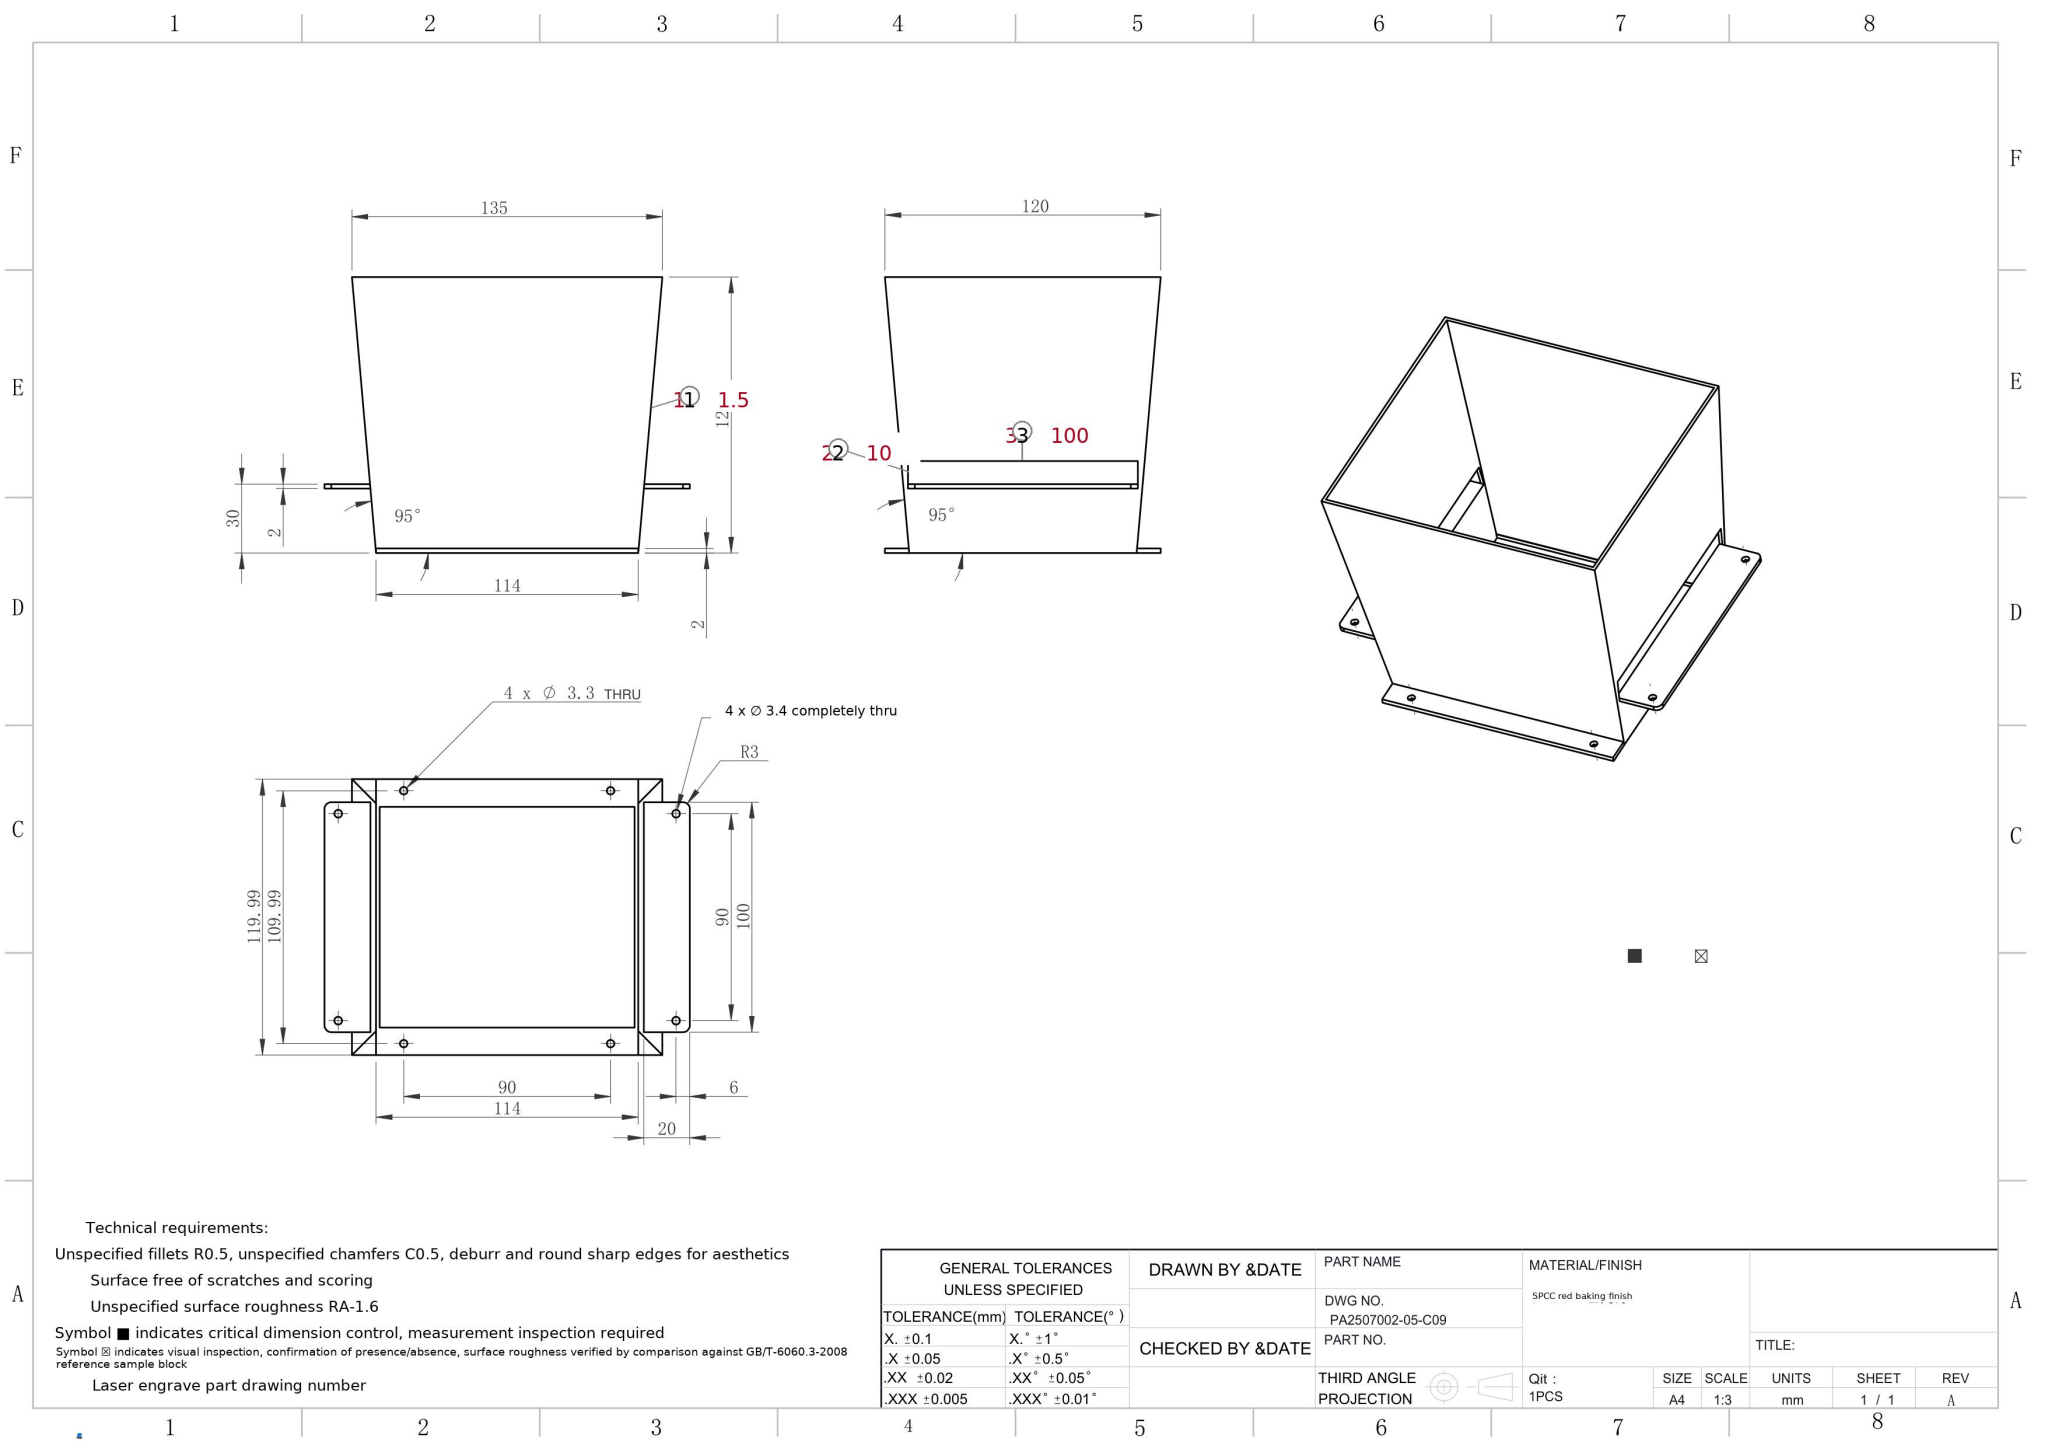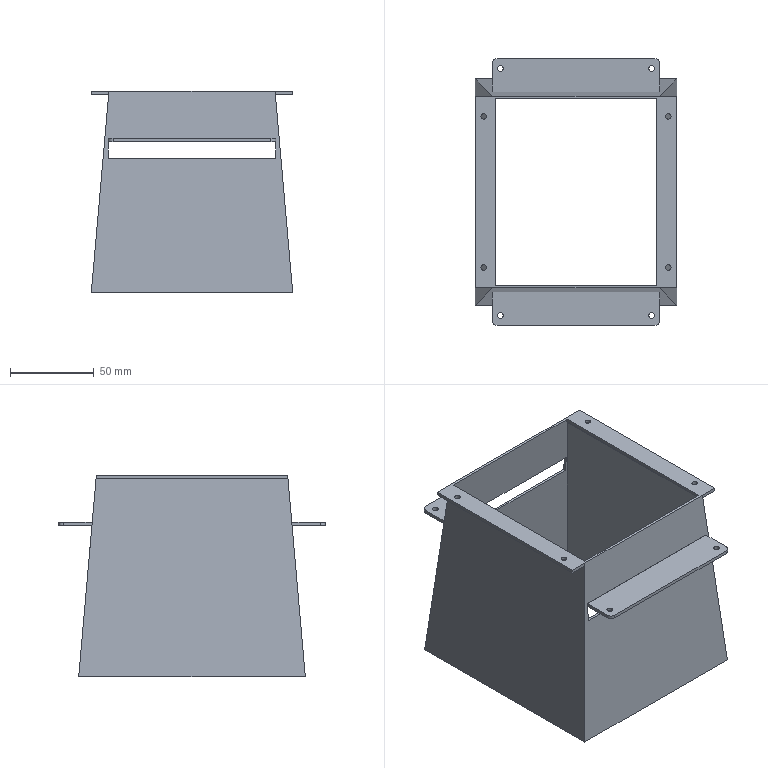Part | SolidWorks | mm | material SPCC red baking finish | 1 solid | 60 faces | box 120 x 159 x 120 mm | volume 93073 mm3 | plane 40 | cylinder 20 | commonest cylinder face diameters 3.4 x8 3.3 x8 6 x4
build123d program:
from build123d import *

# Parameters (mm, degrees)
SKETCH1_W                    = 120
SKETCH1_H                    = 135
BOSS_EXTRUDE1_DEPTH          = 120
BOSS_EXTRUDE1_TAPER          = 5
SHELL1_T                     = -1.5
SKETCH4_W                    = 12
SKETCH4_H                    = 114.003
BOSS_EXTRUDE2_DEPTH          = 2
M4_TAPPED_HOLE_DRILL_1_D     = 3.3
M4_TAPPED_HOLE_DRILL_1_DEPTH = 2
CUT_EXTRUDE3_DEPTH           = 151.187
CUT_EXTRUDE3_DEPTH_BACK      = 151.187
SKETCH7_W                    = 100
SKETCH7_H                    = 10
BOSS_EXTRUDE3_START          = 59.5
SKETCH8_W                    = 100
SKETCH8_H                    = 2
BOSS_EXTRUDE3_DEPTH          = 20
FILLET2_R                    = 3
M3_CLEARANCE_HOLE_1_D        = 3.4


with BuildPart() as part:
    # Sketch1 → Boss-Extrude1 (new body)
    with BuildSketch(Plane.XY):
        Rectangle(SKETCH1_W, SKETCH1_H)
    extrude(amount=BOSS_EXTRUDE1_DEPTH, taper=BOSS_EXTRUDE1_TAPER)

    # Shell1
    shell1_openings = [part.faces().sort_by_distance(p)[0] for p in [
        (0, 0, 120),
        (0, 0, 0),
    ]]
    offset(amount=SHELL1_T, openings=shell1_openings, kind=Kind.INTERSECTION)

    # Sketch4 → Boss-Extrude2 (add)
    with BuildSketch(Plane.XY.offset(120)):
        with Locations((53.996, 0)):
            Rectangle(SKETCH4_W, SKETCH4_H)
        with Locations((-53.996, 0)):
            Rectangle(SKETCH4_W, SKETCH4_H)
    extrude(amount=-BOSS_EXTRUDE2_DEPTH)

    # M4 Tapped Hole Drill 1
    with Locations(Plane.XY.offset(120)):
        with Locations((54.996, -45.001), (54.996, 45.001), (-54.996, 45.001), (-54.996, -45.001)):
            Hole(M4_TAPPED_HOLE_DRILL_1_D / 2, depth=M4_TAPPED_HOLE_DRILL_1_DEPTH)

    # Sketch7 → Cut-Extrude3 (cut, two sides: drawn at the far end of the back side and taken through both)
    with BuildSketch(Plane(origin=(0, 0, 0), x_dir=(1, 0, 0), z_dir=(0, 1, 0)).offset(-CUT_EXTRUDE3_DEPTH_BACK)):
        with Locations((0, -85)):
            Rectangle(SKETCH7_W, SKETCH7_H)
    extrude(amount=CUT_EXTRUDE3_DEPTH + CUT_EXTRUDE3_DEPTH_BACK, mode=Mode.SUBTRACT)

    # Sketch8 → Boss-Extrude3 (add)
    with BuildSketch(Plane(origin=(0, 0, 0), x_dir=(1, 0, 0), z_dir=(0, 1, 0)).offset(BOSS_EXTRUDE3_START)):
        with Locations((0, -91)):
            Rectangle(SKETCH8_W, SKETCH8_H)
    boss_extrude3 = extrude(amount=BOSS_EXTRUDE3_DEPTH)

    # Mirror3: Boss-Extrude3 across plane
    add(boss_extrude3.mirror(Plane.ZX))

    # Fillet2
    fillet2_edges = [part.edges().sort_by_distance(p)[0] for p in [
        (50, 79.5, 91),
        (-50, 79.5, 91),
        (50, -79.5, 91),
        (-50, -79.5, 91),
    ]]
    fillet(fillet2_edges, radius=FILLET2_R)

    # M3 Clearance Hole 1 (through all)
    with Locations(Plane.XY.offset(92)):
        with Locations((-45, -73.5), (45, -73.5), (-45, 73.5), (45, 73.5)):
            Hole(M3_CLEARANCE_HOLE_1_D / 2)


solid = part.part